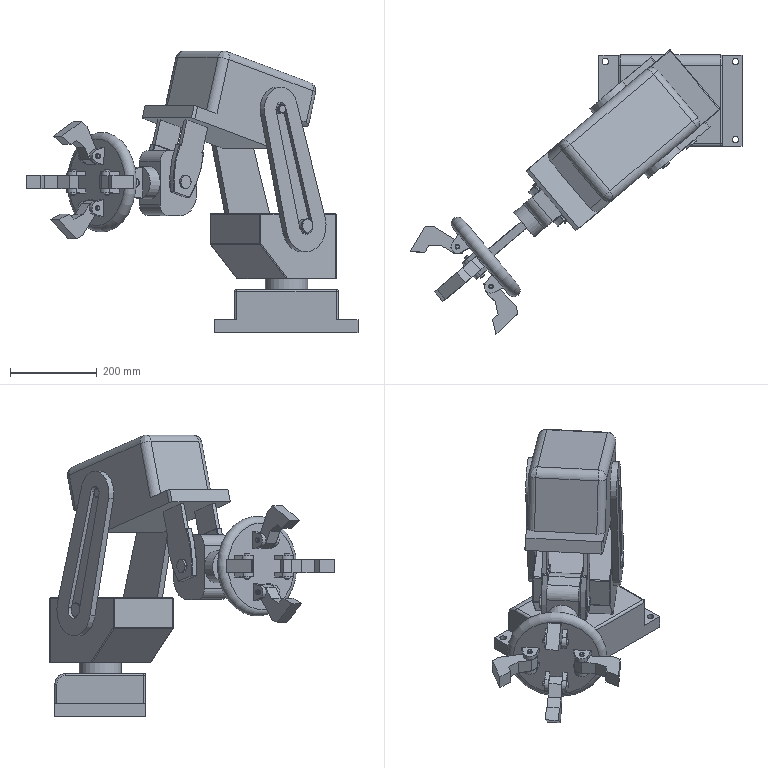Assembly | NX | mm | 18 component files | 25 solids | 522 faces | box 765.41 x 655.18 x 649.88 mm | volume 24426516 mm3 | plane 345 | cylinder 104 | cone 34 | spline 20 | torus 11 | sphere 8 | commonest cylinder face diameters 10 x23 4 x21 30 x16 40 x8 20 x7 100 x4 36 x4 410 x4
Bill of materials:
unnamed part 1 | 1 |  | Disc-shaped body with a rounded, torus-like rim, joined by a tapered arm and short cylindrical boss to a rounded rectangular block that has a through-hole. Small tabs with holes stick out from the back face of the disc.
unnamed part 2 | 1 |  | Slender straight rod with a round shaft. Each end has a slightly larger faceted, roughly hexagonal collar with chamfered edges.
unnamed part 3 | 1 |  | Rectangular block with one corner cut off at an angle, giving a five-sided profile, plus one small round hole on a side face.
unnamed part 4 | 2 |  | Thin flat link bar with rounded ends and one hole near each end. The two holes appear to be different sizes.
unnamed part 5 | 1 |  | Housing-like block: a raised rectangular body with rounded edges on top of a wider flat base plate. The base has four corner holes and the top face has a large round opening.
unnamed part 6 | 1 |  | Plain solid cylinder with flat end faces. Its height and diameter look broadly similar.
unnamed part 7 | 1 |  | Short, fairly thick rod with a round shaft and a faceted, hex-like collar with chamfered edges at each end.
unnamed part 8 | 4 |  | Slender rod with a round shaft and faceted collars at both ends. Each end face shows a smaller circular inner face.
unnamed part 9 | 1 |  | Rectangular cover-like body with rounded edges. Along one side, a flange or step carries two downward-hanging tabs, each with a hole near its tip. There is a curved notch in one side wall and a small hole in a side face.
unnamed part 10 | 4 |  | Flat thick plate, irregularly shaped, roughly like a bent arm or boomerang. A narrow end lobe carries a single round through-hole.
unnamed part 11 | 1 |  | Very slender long rod with a round shaft and small faceted, chamfered collars at both ends.
Mates:
1. fix | M1002_AGO13_P09_A00757058_P03 1 component
2. fix | M1002_AGO13_P09_A00757058_P03 1 component
3. fix | M1002_AGO13_P09_A00757058_P03 1 component
4. fix | M1002_AGO13_P09_A00757058_P03 1 component
5. touch align | M1002_AGO13_P09_A00757058_P03 1 face | tubogiratorio 1 face
6. distance | M1002_AGO13_P09_A00757058_P03 1 face | tubogiratorio 1 face
7. touch align | tubogiratorio 1 face | baseup 1 face
8. distance | baseup 1 face | tubogiratorio 1 face
9. touch align | M1002_AGO13_P09_757058_P02 2 face | baseup 1 face
10. touch align | M1002_AGO13_P09_757058_P02 2 face | baseup 1 face
11. touch align | M1002_AGO13_P09_757058_P02 1 face | baseup 1 face
12. touch align | M1002_AGO13_P09_757058_P02 1 face | baseup 1 face
13. touch align | M1002_AGO13_P09_757058_P02 2 face | bota 1 face
14. touch align | M1002_AGO13_P09_757058_P02 2 face | bota 1 face
15. touch align | M1002_AGO13_P09_757058_P02 1 face | bota 1 face
16. touch align | basepinzas 1 face | bota 1 face
17. touch align | basepinzas 1 face | bota 1 face
18. touch align | perno3 1 face | baseup 1 face
19. distance | M1002_AGO13_P09_757058_P02 1 face | perno3 1 edge
20. touch align | perno2 1 face | basepinzas 1 face
21. distance | bota 1 face | perno2 1 edge
22. touch align | perno4 1 face | bota 1 face
23. distance | M1002_AGO13_P09_757058_P02 1 face | perno4 1 edge
24. touch align | perno 4 face | basepinzas 1 face
25. distance | basepinzas 1 face | perno 4 edge
26. touch align | perno 3 face | basepinzas 1 face
27. distance | basepinzas 1 face | perno 3 edge
28. touch align | perno 2 face | basepinzas 1 face
29. touch align | perno 1 face | basepinzas 1 face
30. distance | basepinzas 1 face | perno 1 edge
31. touch align | M1002_AGO13_P09_757058_P01 4 face | basepinzas 1 face
32. touch align | M1002_AGO13_P09_757058_P01 4 face | basepinzas 1 face
33. touch align | M1002_AGO13_P09_757058_P01 1 face | basepinzas 1 face
34. touch align | basepinzas 1 face | M1002_AGO13_P09_757058_P01 1 face
35. touch align | M1002_AGO13_P09_757058_P01 2 face | basepinzas 1 face
36. touch align | M1002_AGO13_P09_757058_P01 2 face | basepinzas 1 face
37. touch align | M1002_AGO13_P09_757058_P01 3 face | basepinzas 1 face
38. touch align | M1002_AGO13_P09_757058_P01 3 face | basepinzas 1 face